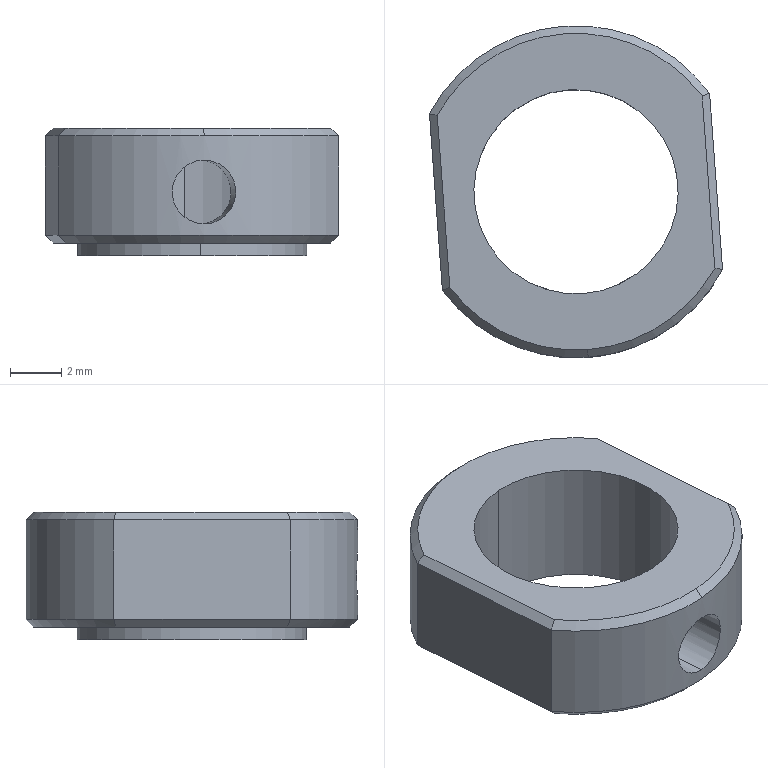Component | SolidWorks | MotorAssemblyWhen2-1_M8Nut2-1 | 1 solid | 24 faces | box 11.48 x 13 x 5 mm | volume 320 mm3 | cylinder 9 | plane 9 | cone 6 | commonest cylinder face diameters 13 x3 8 x2 2.5 x2 9 x2
STEP:
#1=COLOUR_RGB('',0.7922,0.8196,0.9333);
#2=FILL_AREA_STYLE_COLOUR('',#1);
#3=FILL_AREA_STYLE('',(#2));
#4=SURFACE_STYLE_FILL_AREA(#3);
#5=SURFACE_SIDE_STYLE('',(#4));
#6=SURFACE_STYLE_USAGE(.BOTH.,#5);
#7=PRESENTATION_STYLE_ASSIGNMENT((#6));
#8=CARTESIAN_POINT('',(-1.98,5.492,-5.202));
#9=VERTEX_POINT('',#8);
#10=CARTESIAN_POINT('',(-1.957,5.178,-5.202));
#11=VERTEX_POINT('',#10);
#12=CARTESIAN_POINT('',(-1.969,5.335,-5.202));
#13=DIRECTION('',(-0.,0.,-1.));
#14=DIRECTION('',(0.07337,-0.9973,0.));
#15=AXIS2_PLACEMENT_3D('',#12,#13,#14);
#16=CIRCLE('',#15,0.1575);
#17=EDGE_CURVE('',#9,#11,#16,.T.);
#18=ORIENTED_EDGE('',*,*,#17,.F.);
#19=CARTESIAN_POINT('',(-1.98,5.492,-5.398));
#20=VERTEX_POINT('',#19);
#21=CARTESIAN_POINT('',(-1.98,5.492,-5.202));
#22=DIRECTION('',(-0.,0.,-1.));
#23=VECTOR('',#22,39.37);
#24=LINE('',#21,#23);
#25=EDGE_CURVE('',#9,#20,#24,.T.);
#26=ORIENTED_EDGE('',*,*,#25,.T.);
#27=CARTESIAN_POINT('',(-1.957,5.178,-5.398));
#28=VERTEX_POINT('',#27);
#29=CARTESIAN_POINT('',(-1.969,5.335,-5.398));
#30=DIRECTION('',(-0.,0.,-1.));
#31=DIRECTION('',(0.07337,-0.9973,0.));
#32=AXIS2_PLACEMENT_3D('',#29,#30,#31);
#33=CIRCLE('',#32,0.1575);
#34=EDGE_CURVE('',#20,#28,#33,.T.);
#35=ORIENTED_EDGE('',*,*,#34,.T.);
#36=CARTESIAN_POINT('',(-1.957,5.178,-5.349));
#37=VERTEX_POINT('',#36);
#38=CARTESIAN_POINT('',(-1.957,5.178,-5.202));
#39=DIRECTION('',(-0.,0.,-1.));
#40=VECTOR('',#39,39.37);
#41=LINE('',#38,#40);
#42=EDGE_CURVE('',#37,#28,#41,.T.);
#43=ORIENTED_EDGE('',*,*,#42,.F.);
#44=CARTESIAN_POINT('',(-1.957,5.178,-5.251));
#45=VERTEX_POINT('',#44);
#46=CARTESIAN_POINT('',(-1.957,5.178,-5.251));
#47=CARTESIAN_POINT('',(-1.95,5.178,-5.251));
#48=CARTESIAN_POINT('',(-1.944,5.179,-5.252));
#49=CARTESIAN_POINT('',(-1.932,5.181,-5.257));
#50=CARTESIAN_POINT('',(-1.927,5.183,-5.261));
#51=CARTESIAN_POINT('',(-1.918,5.185,-5.27));
#52=CARTESIAN_POINT('',(-1.915,5.187,-5.275));
#53=CARTESIAN_POINT('',(-1.91,5.189,-5.287));
#54=CARTESIAN_POINT('',(-1.908,5.189,-5.294));
#55=CARTESIAN_POINT('',(-1.908,5.189,-5.303));
#56=CARTESIAN_POINT('',(-1.909,5.189,-5.307));
#57=CARTESIAN_POINT('',(-1.91,5.188,-5.313));
#58=CARTESIAN_POINT('',(-1.911,5.188,-5.316));
#59=CARTESIAN_POINT('',(-1.915,5.187,-5.325));
#60=CARTESIAN_POINT('',(-1.918,5.185,-5.33));
#61=CARTESIAN_POINT('',(-1.925,5.183,-5.337));
#62=CARTESIAN_POINT('',(-1.927,5.183,-5.339));
#63=CARTESIAN_POINT('',(-1.932,5.181,-5.343));
#64=CARTESIAN_POINT('',(-1.935,5.181,-5.344));
#65=CARTESIAN_POINT('',(-1.944,5.179,-5.348));
#66=CARTESIAN_POINT('',(-1.951,5.178,-5.349));
#67=CARTESIAN_POINT('',(-1.957,5.178,-5.349));
#68=B_SPLINE_CURVE_WITH_KNOTS('',3,(#46,#47,#48,#49,#50,#51,#52,#53,#54,#55,#56,#57,#58,#59,#60,#61,#62,#63,#64,#65,#66,#67),.UNSPECIFIED.,.F.,.F.,(4,2,2,2,2,2,2,2,2,2,4),(0.,0.0004916,0.0009832,0.001475,0.001966,0.002212,0.002458,0.00295,0.003195,0.003441,0.003933),.UNSPECIFIED.);
#69=EDGE_CURVE('',#45,#37,#68,.T.);
#70=ORIENTED_EDGE('',*,*,#69,.F.);
#71=CARTESIAN_POINT('',(-1.957,5.178,-5.202));
#72=DIRECTION('',(-0.,0.,-1.));
#73=VECTOR('',#72,39.37);
#74=LINE('',#71,#73);
#75=EDGE_CURVE('',#11,#45,#74,.T.);
#76=ORIENTED_EDGE('',*,*,#75,.F.);
#77=EDGE_LOOP('',(#18,#26,#35,#43,#70,#76));
#78=FACE_OUTER_BOUND('',#77,.T.);
#79=CARTESIAN_POINT('',(-1.969,5.335,-5.202));
#80=DIRECTION('',(-0.,0.,-1.));
#81=DIRECTION('',(0.07337,-0.9973,0.));
#82=AXIS2_PLACEMENT_3D('',#79,#80,#81);
#83=CYLINDRICAL_SURFACE('',#82,0.1575);
#84=ADVANCED_FACE('',(#78),#83,.F.);
#85=CARTESIAN_POINT('',(-1.986,5.578,-5.379));
#86=VERTEX_POINT('',#85);
#87=CARTESIAN_POINT('',(-1.774,5.482,-5.379));
#88=VERTEX_POINT('',#87);
#89=CARTESIAN_POINT('',(-1.969,5.335,-5.379));
#90=DIRECTION('',(-0.,0.,-1.));
#91=DIRECTION('',(0.07337,-0.9973,0.));
#92=AXIS2_PLACEMENT_3D('',#89,#90,#91);
#93=CIRCLE('',#92,0.2441);
#94=EDGE_CURVE('',#86,#88,#93,.T.);
#95=ORIENTED_EDGE('',*,*,#94,.F.);
#96=CARTESIAN_POINT('',(-1.987,5.59,-5.367));
#97=VERTEX_POINT('',#96);
#98=CARTESIAN_POINT('',(-1.987,5.59,-5.367));
#99=DIRECTION('',(-0.05188,0.7052,0.7071));
#100=VECTOR('',#99,39.37);
#101=LINE('',#98,#100);
#102=EDGE_CURVE('',#86,#97,#101,.T.);
#103=ORIENTED_EDGE('',*,*,#102,.T.);
#104=CARTESIAN_POINT('',(-1.763,5.487,-5.367));
#105=VERTEX_POINT('',#104);
#106=CARTESIAN_POINT('',(-1.969,5.335,-5.367));
#107=DIRECTION('',(0.,-0.,1.));
#108=DIRECTION('',(0.07337,-0.9973,0.));
#109=AXIS2_PLACEMENT_3D('',#106,#107,#108);
#110=CIRCLE('',#109,0.2559);
#111=EDGE_CURVE('',#105,#97,#110,.T.);
#112=ORIENTED_EDGE('',*,*,#111,.F.);
#113=CARTESIAN_POINT('',(-1.774,5.482,-5.379));
#114=CARTESIAN_POINT('',(-1.77,5.484,-5.375));
#115=CARTESIAN_POINT('',(-1.766,5.485,-5.371));
#116=CARTESIAN_POINT('',(-1.763,5.487,-5.367));
#117=B_SPLINE_CURVE_WITH_KNOTS('',3,(#113,#114,#115,#116),.UNSPECIFIED.,.F.,.F.,(4,4),(0.,0.0004332),.UNSPECIFIED.);
#118=EDGE_CURVE('',#88,#105,#117,.T.);
#119=ORIENTED_EDGE('',*,*,#118,.F.);
#120=EDGE_LOOP('',(#95,#103,#112,#119));
#121=FACE_OUTER_BOUND('',#120,.T.);
#122=CARTESIAN_POINT('',(-1.969,5.335,-5.367));
#123=DIRECTION('',(0.,-0.,1.));
#124=DIRECTION('',(-0.07337,0.9973,0.));
#125=AXIS2_PLACEMENT_3D('',#122,#123,#124);
#126=CONICAL_SURFACE('',#125,0.2559,0.7854);
#127=ADVANCED_FACE('',(#121),#126,.T.);
#128=CARTESIAN_POINT('',(-1.951,5.091,-5.202));
#129=VERTEX_POINT('',#128);
#130=CARTESIAN_POINT('',(-1.755,5.217,-5.202));
#131=VERTEX_POINT('',#130);
#132=CARTESIAN_POINT('',(-1.969,5.335,-5.202));
#133=DIRECTION('',(0.,-0.,1.));
#134=DIRECTION('',(0.07337,-0.9973,0.));
#135=AXIS2_PLACEMENT_3D('',#132,#133,#134);
#136=CIRCLE('',#135,0.2441);
#137=EDGE_CURVE('',#129,#131,#136,.T.);
#138=ORIENTED_EDGE('',*,*,#137,.F.);
#139=CARTESIAN_POINT('',(-1.95,5.079,-5.213));
#140=VERTEX_POINT('',#139);
#141=CARTESIAN_POINT('',(-1.95,5.079,-5.213));
#142=DIRECTION('',(0.05188,-0.7052,-0.7071));
#143=VECTOR('',#142,39.37);
#144=LINE('',#141,#143);
#145=EDGE_CURVE('',#129,#140,#144,.T.);
#146=ORIENTED_EDGE('',*,*,#145,.T.);
#147=CARTESIAN_POINT('',(-1.743,5.215,-5.213));
#148=VERTEX_POINT('',#147);
#149=CARTESIAN_POINT('',(-1.969,5.335,-5.213));
#150=DIRECTION('',(-0.,0.,-1.));
#151=DIRECTION('',(0.07337,-0.9973,0.));
#152=AXIS2_PLACEMENT_3D('',#149,#150,#151);
#153=CIRCLE('',#152,0.2559);
#154=EDGE_CURVE('',#148,#140,#153,.T.);
#155=ORIENTED_EDGE('',*,*,#154,.F.);
#156=CARTESIAN_POINT('',(-1.743,5.215,-5.213));
#157=CARTESIAN_POINT('',(-1.747,5.215,-5.209));
#158=CARTESIAN_POINT('',(-1.751,5.216,-5.206));
#159=CARTESIAN_POINT('',(-1.755,5.217,-5.202));
#160=B_SPLINE_CURVE_WITH_KNOTS('',3,(#156,#157,#158,#159),.UNSPECIFIED.,.F.,.F.,(4,4),(0.,0.0004332),.UNSPECIFIED.);
#161=EDGE_CURVE('',#148,#131,#160,.T.);
#162=ORIENTED_EDGE('',*,*,#161,.T.);
#163=EDGE_LOOP('',(#138,#146,#155,#162));
#164=FACE_OUTER_BOUND('',#163,.T.);
#165=CARTESIAN_POINT('',(-1.969,5.335,-5.213));
#166=DIRECTION('',(-0.,0.,-1.));
#167=DIRECTION('',(0.07337,-0.9973,0.));
#168=AXIS2_PLACEMENT_3D('',#165,#166,#167);
#169=CONICAL_SURFACE('',#168,0.2559,0.7854);
#170=ADVANCED_FACE('',(#164),#169,.T.);
#171=ORIENTED_EDGE('',*,*,#111,.T.);
#172=CARTESIAN_POINT('',(-1.987,5.59,-5.213));
#173=VERTEX_POINT('',#172);
#174=CARTESIAN_POINT('',(-1.987,5.59,-5.398));
#175=DIRECTION('',(0.,-0.,1.));
#176=VECTOR('',#175,39.37);
#177=LINE('',#174,#176);
#178=EDGE_CURVE('',#97,#173,#177,.T.);
#179=ORIENTED_EDGE('',*,*,#178,.T.);
#180=CARTESIAN_POINT('',(-1.763,5.487,-5.213));
#181=VERTEX_POINT('',#180);
#182=CARTESIAN_POINT('',(-1.969,5.335,-5.213));
#183=DIRECTION('',(-0.,0.,-1.));
#184=DIRECTION('',(0.07337,-0.9973,0.));
#185=AXIS2_PLACEMENT_3D('',#182,#183,#184);
#186=CIRCLE('',#185,0.2559);
#187=EDGE_CURVE('',#173,#181,#186,.T.);
#188=ORIENTED_EDGE('',*,*,#187,.T.);
#189=CARTESIAN_POINT('',(-1.763,5.487,-5.202));
#190=DIRECTION('',(0.,-0.,1.));
#191=VECTOR('',#190,39.37);
#192=LINE('',#189,#191);
#193=EDGE_CURVE('',#105,#181,#192,.T.);
#194=ORIENTED_EDGE('',*,*,#193,.F.);
#195=EDGE_LOOP('',(#171,#179,#188,#194));
#196=FACE_OUTER_BOUND('',#195,.T.);
#197=CARTESIAN_POINT('',(-1.969,5.335,-5.398));
#198=DIRECTION('',(0.,-0.,1.));
#199=DIRECTION('',(-0.07337,0.9973,0.));
#200=AXIS2_PLACEMENT_3D('',#197,#198,#199);
#201=CYLINDRICAL_SURFACE('',#200,0.2559);
#202=ADVANCED_FACE('',(#196),#201,.T.);
#203=ORIENTED_EDGE('',*,*,#69,.T.);
#204=CARTESIAN_POINT('',(-1.95,5.079,-5.349));
#205=VERTEX_POINT('',#204);
#206=CARTESIAN_POINT('',(-1.945,5.021,-5.349));
#207=DIRECTION('',(0.07337,-0.9973,-0.));
#208=VECTOR('',#207,39.37);
#209=LINE('',#206,#208);
#210=EDGE_CURVE('',#37,#205,#209,.T.);
#211=ORIENTED_EDGE('',*,*,#210,.T.);
#212=CARTESIAN_POINT('',(-1.95,5.079,-5.251));
#213=VERTEX_POINT('',#212);
#214=CARTESIAN_POINT('',(-1.95,5.079,-5.251));
#215=CARTESIAN_POINT('',(-1.943,5.08,-5.251));
#216=CARTESIAN_POINT('',(-1.937,5.081,-5.252));
#217=CARTESIAN_POINT('',(-1.925,5.082,-5.257));
#218=CARTESIAN_POINT('',(-1.92,5.083,-5.261));
#219=CARTESIAN_POINT('',(-1.911,5.085,-5.27));
#220=CARTESIAN_POINT('',(-1.907,5.086,-5.275));
#221=CARTESIAN_POINT('',(-1.902,5.087,-5.287));
#222=CARTESIAN_POINT('',(-1.901,5.088,-5.294));
#223=CARTESIAN_POINT('',(-1.901,5.088,-5.303));
#224=CARTESIAN_POINT('',(-1.901,5.088,-5.306));
#225=CARTESIAN_POINT('',(-1.903,5.087,-5.313));
#226=CARTESIAN_POINT('',(-1.903,5.087,-5.316));
#227=CARTESIAN_POINT('',(-1.907,5.086,-5.325));
#228=CARTESIAN_POINT('',(-1.911,5.085,-5.33));
#229=CARTESIAN_POINT('',(-1.92,5.083,-5.339));
#230=CARTESIAN_POINT('',(-1.925,5.082,-5.343));
#231=CARTESIAN_POINT('',(-1.937,5.081,-5.348));
#232=CARTESIAN_POINT('',(-1.943,5.08,-5.349));
#233=CARTESIAN_POINT('',(-1.95,5.079,-5.349));
#234=B_SPLINE_CURVE_WITH_KNOTS('',3,(#214,#215,#216,#217,#218,#219,#220,#221,#222,#223,#224,#225,#226,#227,#228,#229,#230,#231,#232,#233),.UNSPECIFIED.,.F.,.F.,(4,2,2,2,2,2,2,2,2,4),(0.003916,0.004406,0.004895,0.005385,0.005874,0.006119,0.006364,0.006853,0.007343,0.007832),.UNSPECIFIED.);
#235=EDGE_CURVE('',#213,#205,#234,.T.);
#236=ORIENTED_EDGE('',*,*,#235,.F.);
#237=CARTESIAN_POINT('',(-1.945,5.021,-5.251));
#238=DIRECTION('',(0.07337,-0.9973,-0.));
#239=VECTOR('',#238,39.37);
#240=LINE('',#237,#239);
#241=EDGE_CURVE('',#45,#213,#240,.T.);
#242=ORIENTED_EDGE('',*,*,#241,.F.);
#243=EDGE_LOOP('',(#203,#211,#236,#242));
#244=FACE_OUTER_BOUND('',#243,.T.);
#245=CARTESIAN_POINT('',(-1.945,5.021,-5.3));
#246=DIRECTION('',(0.07337,-0.9973,-0.));
#247=DIRECTION('',(0.,0.,1.));
#248=AXIS2_PLACEMENT_3D('',#245,#246,#247);
#249=CYLINDRICAL_SURFACE('',#248,0.04921);
#250=ADVANCED_FACE('',(#244),#249,.F.);
#251=CARTESIAN_POINT('',(-1.982,5.511,-5.379));
#252=VERTEX_POINT('',#251);
#253=CARTESIAN_POINT('',(-1.956,5.158,-5.379));
#254=VERTEX_POINT('',#253);
#255=CARTESIAN_POINT('',(-1.969,5.335,-5.379));
#256=DIRECTION('',(0.,-0.,1.));
#257=DIRECTION('',(0.07337,-0.9973,0.));
#258=AXIS2_PLACEMENT_3D('',#255,#256,#257);
#259=CIRCLE('',#258,0.1772);
#260=EDGE_CURVE('',#252,#254,#259,.T.);
#261=ORIENTED_EDGE('',*,*,#260,.F.);
#262=CARTESIAN_POINT('',(-1.982,5.511,-5.398));
#263=VERTEX_POINT('',#262);
#264=CARTESIAN_POINT('',(-1.982,5.511,-5.379));
#265=DIRECTION('',(-0.,0.,-1.));
#266=VECTOR('',#265,39.37);
#267=LINE('',#264,#266);
#268=EDGE_CURVE('',#252,#263,#267,.T.);
#269=ORIENTED_EDGE('',*,*,#268,.T.);
#270=CARTESIAN_POINT('',(-1.956,5.158,-5.398));
#271=VERTEX_POINT('',#270);
#272=CARTESIAN_POINT('',(-1.969,5.335,-5.398));
#273=DIRECTION('',(-0.,0.,-1.));
#274=DIRECTION('',(0.07337,-0.9973,0.));
#275=AXIS2_PLACEMENT_3D('',#272,#273,#274);
#276=CIRCLE('',#275,0.1772);
#277=EDGE_CURVE('',#271,#263,#276,.T.);
#278=ORIENTED_EDGE('',*,*,#277,.F.);
#279=CARTESIAN_POINT('',(-1.956,5.158,-5.379));
#280=DIRECTION('',(-0.,0.,-1.));
#281=VECTOR('',#280,39.37);
#282=LINE('',#279,#281);
#283=EDGE_CURVE('',#254,#271,#282,.T.);
#284=ORIENTED_EDGE('',*,*,#283,.F.);
#285=EDGE_LOOP('',(#261,#269,#278,#284));
#286=FACE_OUTER_BOUND('',#285,.T.);
#287=CARTESIAN_POINT('',(-1.969,5.335,-5.379));
#288=DIRECTION('',(-0.,0.,-1.));
#289=DIRECTION('',(0.07337,-0.9973,0.));
#290=AXIS2_PLACEMENT_3D('',#287,#288,#289);
#291=CYLINDRICAL_SURFACE('',#290,0.1772);
#292=ADVANCED_FACE('',(#286),#291,.T.);
#293=CARTESIAN_POINT('',(-1.969,5.335,-5.202));
#294=DIRECTION('',(-0.,0.,-1.));
#295=DIRECTION('',(0.07337,-0.9973,0.));
#296=AXIS2_PLACEMENT_3D('',#293,#294,#295);
#297=CIRCLE('',#296,0.1575);
#298=EDGE_CURVE('',#11,#9,#297,.T.);
#299=ORIENTED_EDGE('',*,*,#298,.T.);
#300=ORIENTED_EDGE('',*,*,#17,.T.);
#301=EDGE_LOOP('',(#299,#300));
#302=FACE_BOUND('',#301,.T.);
#303=CARTESIAN_POINT('',(-1.774,5.482,-5.202));
#304=VERTEX_POINT('',#303);
#305=CARTESIAN_POINT('',(-2.182,5.452,-5.202));
#306=VERTEX_POINT('',#305);
#307=CARTESIAN_POINT('',(-1.969,5.335,-5.202));
#308=DIRECTION('',(0.,-0.,1.));
#309=DIRECTION('',(0.07337,-0.9973,0.));
#310=AXIS2_PLACEMENT_3D('',#307,#308,#309);
#311=CIRCLE('',#310,0.2441);
#312=EDGE_CURVE('',#304,#306,#311,.T.);
#313=ORIENTED_EDGE('',*,*,#312,.T.);
#314=CARTESIAN_POINT('',(-2.163,5.187,-5.202));
#315=VERTEX_POINT('',#314);
#316=CARTESIAN_POINT('',(-2.163,5.184,-5.202));
#317=DIRECTION('',(0.07337,-0.9973,-0.));
#318=VECTOR('',#317,39.37);
#319=LINE('',#316,#318);
#320=EDGE_CURVE('',#306,#315,#319,.T.);
#321=ORIENTED_EDGE('',*,*,#320,.T.);
#322=CARTESIAN_POINT('',(-1.969,5.335,-5.202));
#323=DIRECTION('',(0.,-0.,1.));
#324=DIRECTION('',(0.07337,-0.9973,0.));
#325=AXIS2_PLACEMENT_3D('',#322,#323,#324);
#326=CIRCLE('',#325,0.2441);
#327=EDGE_CURVE('',#315,#129,#326,.T.);
#328=ORIENTED_EDGE('',*,*,#327,.T.);
#329=ORIENTED_EDGE('',*,*,#137,.T.);
#330=CARTESIAN_POINT('',(-1.774,5.486,-5.202));
#331=DIRECTION('',(-0.07337,0.9973,0.));
#332=VECTOR('',#331,39.37);
#333=LINE('',#330,#332);
#334=EDGE_CURVE('',#131,#304,#333,.T.);
#335=ORIENTED_EDGE('',*,*,#334,.T.);
#336=EDGE_LOOP('',(#313,#321,#328,#329,#335));
#337=FACE_OUTER_BOUND('',#336,.T.);
#338=CARTESIAN_POINT('',(-1.969,5.335,-5.202));
#339=DIRECTION('',(-0.,0.,-1.));
#340=DIRECTION('',(0.07337,-0.9973,-0.));
#341=AXIS2_PLACEMENT_3D('',#338,#339,#340);
#342=PLANE('',#341);
#343=ADVANCED_FACE('',(#302,#337),#342,.F.);
#344=ORIENTED_EDGE('',*,*,#193,.T.);
#345=CARTESIAN_POINT('',(-1.743,5.215,-5.213));
#346=DIRECTION('',(0.07337,-0.9973,-0.));
#347=VECTOR('',#346,39.37);
#348=LINE('',#345,#347);
#349=EDGE_CURVE('',#181,#148,#348,.T.);
#350=ORIENTED_EDGE('',*,*,#349,.T.);
#351=CARTESIAN_POINT('',(-1.743,5.215,-5.367));
#352=VERTEX_POINT('',#351);
#353=CARTESIAN_POINT('',(-1.743,5.215,-5.202));
#354=DIRECTION('',(-0.,0.,-1.));
#355=VECTOR('',#354,39.37);
#356=LINE('',#353,#355);
#357=EDGE_CURVE('',#148,#352,#356,.T.);
#358=ORIENTED_EDGE('',*,*,#357,.T.);
#359=CARTESIAN_POINT('',(-1.781,5.743,-5.367));
#360=DIRECTION('',(-0.07337,0.9973,0.));
#361=VECTOR('',#360,39.37);
#362=LINE('',#359,#361);
#363=EDGE_CURVE('',#352,#105,#362,.T.);
#364=ORIENTED_EDGE('',*,*,#363,.T.);
#365=EDGE_LOOP('',(#344,#350,#358,#364));
#366=FACE_OUTER_BOUND('',#365,.T.);
#367=CARTESIAN_POINT('',(-1.781,5.743,-5.202));
#368=DIRECTION('',(0.9973,0.07337,0.));
#369=DIRECTION('',(0.,-0.,1.));
#370=AXIS2_PLACEMENT_3D('',#367,#368,#369);
#371=PLANE('',#370);
#372=ADVANCED_FACE('',(#366),#371,.T.);
#373=ORIENTED_EDGE('',*,*,#178,.F.);
#374=CARTESIAN_POINT('',(-2.194,5.455,-5.367));
#375=VERTEX_POINT('',#374);
#376=CARTESIAN_POINT('',(-1.969,5.335,-5.367));
#377=DIRECTION('',(0.,-0.,1.));
#378=DIRECTION('',(0.07337,-0.9973,0.));
#379=AXIS2_PLACEMENT_3D('',#376,#377,#378);
#380=CIRCLE('',#379,0.2559);
#381=EDGE_CURVE('',#97,#375,#380,.T.);
#382=ORIENTED_EDGE('',*,*,#381,.T.);
#383=CARTESIAN_POINT('',(-2.194,5.455,-5.213));
#384=VERTEX_POINT('',#383);
#385=CARTESIAN_POINT('',(-2.194,5.455,-5.398));
#386=DIRECTION('',(0.,-0.,1.));
#387=VECTOR('',#386,39.37);
#388=LINE('',#385,#387);
#389=EDGE_CURVE('',#375,#384,#388,.T.);
#390=ORIENTED_EDGE('',*,*,#389,.T.);
#391=CARTESIAN_POINT('',(-1.969,5.335,-5.213));
#392=DIRECTION('',(-0.,0.,-1.));
#393=DIRECTION('',(0.07337,-0.9973,0.));
#394=AXIS2_PLACEMENT_3D('',#391,#392,#393);
#395=CIRCLE('',#394,0.2559);
#396=EDGE_CURVE('',#384,#173,#395,.T.);
#397=ORIENTED_EDGE('',*,*,#396,.T.);
#398=EDGE_LOOP('',(#373,#382,#390,#397));
#399=FACE_OUTER_BOUND('',#398,.T.);
#400=CARTESIAN_POINT('',(-1.969,5.335,-5.398));
#401=DIRECTION('',(0.,-0.,1.));
#402=DIRECTION('',(-0.07337,0.9973,0.));
#403=AXIS2_PLACEMENT_3D('',#400,#401,#402);
#404=CYLINDRICAL_SURFACE('',#403,0.2559);
#405=ADVANCED_FACE('',(#399),#404,.T.);
#406=CARTESIAN_POINT('',(-2.174,5.183,-5.367));
#407=VERTEX_POINT('',#406);
#408=CARTESIAN_POINT('',(-2.174,5.183,-5.213));
#409=VERTEX_POINT('',#408);
#410=CARTESIAN_POINT('',(-2.174,5.183,-5.202));
#411=DIRECTION('',(0.,-0.,1.));
#412=VECTOR('',#411,39.37);
#413=LINE('',#410,#412);
#414=EDGE_CURVE('',#407,#409,#413,.T.);
#415=ORIENTED_EDGE('',*,*,#414,.T.);
#416=CARTESIAN_POINT('',(-2.194,5.455,-5.213));
#417=DIRECTION('',(-0.07337,0.9973,0.));
#418=VECTOR('',#417,39.37);
#419=LINE('',#416,#418);
#420=EDGE_CURVE('',#409,#384,#419,.T.);
#421=ORIENTED_EDGE('',*,*,#420,.T.);
#422=ORIENTED_EDGE('',*,*,#389,.F.);
#423=CARTESIAN_POINT('',(-2.213,5.711,-5.367));
#424=DIRECTION('',(0.07337,-0.9973,-0.));
#425=VECTOR('',#424,39.37);
#426=LINE('',#423,#425);
#427=EDGE_CURVE('',#375,#407,#426,.T.);
#428=ORIENTED_EDGE('',*,*,#427,.T.);
#429=EDGE_LOOP('',(#415,#421,#422,#428));
#430=FACE_OUTER_BOUND('',#429,.T.);
#431=CARTESIAN_POINT('',(-2.213,5.711,-5.202));
#432=DIRECTION('',(-0.9973,-0.07337,-0.));
#433=DIRECTION('',(-0.,0.,-1.));
#434=AXIS2_PLACEMENT_3D('',#431,#432,#433);
#435=PLANE('',#434);
#436=ADVANCED_FACE('',(#430),#435,.T.);
#437=ORIENTED_EDGE('',*,*,#357,.F.);
#438=ORIENTED_EDGE('',*,*,#154,.T.);
#439=CARTESIAN_POINT('',(-1.969,5.335,-5.213));
#440=DIRECTION('',(-0.,0.,-1.));
#441=DIRECTION('',(0.07337,-0.9973,0.));
#442=AXIS2_PLACEMENT_3D('',#439,#440,#441);
#443=CIRCLE('',#442,0.2559);
#444=EDGE_CURVE('',#140,#409,#443,.T.);
#445=ORIENTED_EDGE('',*,*,#444,.T.);
#446=ORIENTED_EDGE('',*,*,#414,.F.);
#447=CARTESIAN_POINT('',(-1.969,5.335,-5.367));
#448=DIRECTION('',(0.,-0.,1.));
#449=DIRECTION('',(0.07337,-0.9973,0.));
#450=AXIS2_PLACEMENT_3D('',#447,#448,#449);
#451=CIRCLE('',#450,0.2559);
#452=EDGE_CURVE('',#407,#352,#451,.T.);
#453=ORIENTED_EDGE('',*,*,#452,.T.);
#454=EDGE_LOOP('',(#437,#438,#445,#446,#453));
#455=FACE_OUTER_BOUND('',#454,.T.);
#456=ORIENTED_EDGE('',*,*,#235,.T.);
#457=CARTESIAN_POINT('',(-1.95,5.079,-5.349));
#458=CARTESIAN_POINT('',(-1.956,5.079,-5.349));
#459=CARTESIAN_POINT('',(-1.963,5.079,-5.348));
#460=CARTESIAN_POINT('',(-1.975,5.079,-5.343));
#461=CARTESIAN_POINT('',(-1.98,5.079,-5.339));
#462=CARTESIAN_POINT('',(-1.989,5.08,-5.33));
#463=CARTESIAN_POINT('',(-1.993,5.08,-5.325));
#464=CARTESIAN_POINT('',(-1.998,5.08,-5.313));
#465=CARTESIAN_POINT('',(-1.999,5.081,-5.307));
#466=CARTESIAN_POINT('',(-1.999,5.081,-5.297));
#467=CARTESIAN_POINT('',(-1.999,5.081,-5.294));
#468=CARTESIAN_POINT('',(-1.998,5.08,-5.287));
#469=CARTESIAN_POINT('',(-1.997,5.08,-5.284));
#470=CARTESIAN_POINT('',(-1.993,5.08,-5.275));
#471=CARTESIAN_POINT('',(-1.989,5.08,-5.27));
#472=CARTESIAN_POINT('',(-1.98,5.079,-5.261));
#473=CARTESIAN_POINT('',(-1.975,5.079,-5.257));
#474=CARTESIAN_POINT('',(-1.963,5.079,-5.252));
#475=CARTESIAN_POINT('',(-1.956,5.079,-5.251));
#476=CARTESIAN_POINT('',(-1.95,5.079,-5.251));
#477=B_SPLINE_CURVE_WITH_KNOTS('',3,(#457,#458,#459,#460,#461,#462,#463,#464,#465,#466,#467,#468,#469,#470,#471,#472,#473,#474,#475,#476),.UNSPECIFIED.,.F.,.F.,(4,2,2,2,2,2,2,2,2,4),(0.,0.0004895,0.000979,0.001469,0.001958,0.002203,0.002448,0.002937,0.003427,0.003916),.UNSPECIFIED.);
#478=EDGE_CURVE('',#205,#213,#477,.T.);
#479=ORIENTED_EDGE('',*,*,#478,.T.);
#480=EDGE_LOOP('',(#456,#479));
#481=FACE_BOUND('',#480,.T.);
#482=CARTESIAN_POINT('',(-1.969,5.335,-5.398));
#483=DIRECTION('',(0.,-0.,1.));
#484=DIRECTION('',(-0.07337,0.9973,0.));
#485=AXIS2_PLACEMENT_3D('',#482,#483,#484);
#486=CYLINDRICAL_SURFACE('',#485,0.2559);
#487=ADVANCED_FACE('',(#455,#481),#486,.T.);
#488=CARTESIAN_POINT('',(-2.182,5.452,-5.379));
#489=VERTEX_POINT('',#488);
#490=CARTESIAN_POINT('',(-1.969,5.335,-5.379));
#491=DIRECTION('',(-0.,0.,-1.));
#492=DIRECTION('',(0.07337,-0.9973,0.));
#493=AXIS2_PLACEMENT_3D('',#490,#491,#492);
#494=CIRCLE('',#493,0.2441);
#495=EDGE_CURVE('',#489,#86,#494,.T.);
#496=ORIENTED_EDGE('',*,*,#495,.T.);
#497=ORIENTED_EDGE('',*,*,#94,.T.);
#498=CARTESIAN_POINT('',(-1.755,5.217,-5.379));
#499=VERTEX_POINT('',#498);
#500=CARTESIAN_POINT('',(-1.764,5.35,-5.379));
#501=DIRECTION('',(0.07337,-0.9973,-0.));
#502=VECTOR('',#501,39.37);
#503=LINE('',#500,#502);
#504=EDGE_CURVE('',#88,#499,#503,.T.);
#505=ORIENTED_EDGE('',*,*,#504,.T.);
#506=CARTESIAN_POINT('',(-2.163,5.187,-5.379));
#507=VERTEX_POINT('',#506);
#508=CARTESIAN_POINT('',(-1.969,5.335,-5.379));
#509=DIRECTION('',(-0.,0.,-1.));
#510=DIRECTION('',(0.07337,-0.9973,0.));
#511=AXIS2_PLACEMENT_3D('',#508,#509,#510);
#512=CIRCLE('',#511,0.2441);
#513=EDGE_CURVE('',#499,#507,#512,.T.);
#514=ORIENTED_EDGE('',*,*,#513,.T.);
#515=CARTESIAN_POINT('',(-2.173,5.32,-5.379));
#516=DIRECTION('',(-0.07337,0.9973,0.));
#517=VECTOR('',#516,39.37);
#518=LINE('',#515,#517);
#519=EDGE_CURVE('',#507,#489,#518,.T.);
#520=ORIENTED_EDGE('',*,*,#519,.T.);
#521=EDGE_LOOP('',(#496,#497,#505,#514,#520));
#522=FACE_OUTER_BOUND('',#521,.T.);
#523=CARTESIAN_POINT('',(-1.969,5.335,-5.379));
#524=DIRECTION('',(0.,-0.,1.));
#525=DIRECTION('',(0.07337,-0.9973,0.));
#526=AXIS2_PLACEMENT_3D('',#523,#524,#525);
#527=CIRCLE('',#526,0.1772);
#528=EDGE_CURVE('',#254,#252,#527,.T.);
#529=ORIENTED_EDGE('',*,*,#528,.T.);
#530=ORIENTED_EDGE('',*,*,#260,.T.);
#531=EDGE_LOOP('',(#529,#530));
#532=FACE_BOUND('',#531,.T.);
#533=CARTESIAN_POINT('',(-1.969,5.335,-5.379));
#534=DIRECTION('',(-0.,0.,-1.));
#535=DIRECTION('',(0.07337,-0.9973,-0.));
#536=AXIS2_PLACEMENT_3D('',#533,#534,#535);
#537=PLANE('',#536);
#538=ADVANCED_FACE('',(#522,#532),#537,.T.);
#539=ORIENTED_EDGE('',*,*,#210,.F.);
#540=CARTESIAN_POINT('',(-1.957,5.178,-5.349));
#541=CARTESIAN_POINT('',(-1.963,5.177,-5.349));
#542=CARTESIAN_POINT('',(-1.97,5.177,-5.348));
#543=CARTESIAN_POINT('',(-1.982,5.178,-5.343));
#544=CARTESIAN_POINT('',(-1.987,5.178,-5.339));
#545=CARTESIAN_POINT('',(-1.997,5.18,-5.33));
#546=CARTESIAN_POINT('',(-2.,5.18,-5.325));
#547=CARTESIAN_POINT('',(-2.004,5.181,-5.316));
#548=CARTESIAN_POINT('',(-2.005,5.181,-5.313));
#549=CARTESIAN_POINT('',(-2.006,5.182,-5.307));
#550=CARTESIAN_POINT('',(-2.007,5.182,-5.303));
#551=CARTESIAN_POINT('',(-2.007,5.182,-5.294));
#552=CARTESIAN_POINT('',(-2.005,5.181,-5.287));
#553=CARTESIAN_POINT('',(-2.,5.18,-5.275));
#554=CARTESIAN_POINT('',(-1.997,5.18,-5.27));
#555=CARTESIAN_POINT('',(-1.987,5.178,-5.261));
#556=CARTESIAN_POINT('',(-1.982,5.178,-5.257));
#557=CARTESIAN_POINT('',(-1.97,5.177,-5.252));
#558=CARTESIAN_POINT('',(-1.963,5.177,-5.251));
#559=CARTESIAN_POINT('',(-1.957,5.178,-5.251));
#560=B_SPLINE_CURVE_WITH_KNOTS('',3,(#540,#541,#542,#543,#544,#545,#546,#547,#548,#549,#550,#551,#552,#553,#554,#555,#556,#557,#558,#559),.UNSPECIFIED.,.F.,.F.,(4,2,2,2,2,2,2,2,2,4),(0.003933,0.004424,0.004916,0.005407,0.005653,0.005899,0.00639,0.006882,0.007373,0.007865),.UNSPECIFIED.);
#561=EDGE_CURVE('',#37,#45,#560,.T.);
#562=ORIENTED_EDGE('',*,*,#561,.T.);
#563=ORIENTED_EDGE('',*,*,#241,.T.);
#564=ORIENTED_EDGE('',*,*,#478,.F.);
#565=EDGE_LOOP('',(#539,#562,#563,#564));
#566=FACE_OUTER_BOUND('',#565,.T.);
#567=CARTESIAN_POINT('',(-1.945,5.021,-5.3));
#568=DIRECTION('',(0.07337,-0.9973,-0.));
#569=DIRECTION('',(0.,0.,1.));
#570=AXIS2_PLACEMENT_3D('',#567,#568,#569);
#571=CYLINDRICAL_SURFACE('',#570,0.04921);
#572=ADVANCED_FACE('',(#566),#571,.F.);
#573=CARTESIAN_POINT('',(-1.969,5.335,-5.398));
#574=DIRECTION('',(-0.,0.,-1.));
#575=DIRECTION('',(0.07337,-0.9973,0.));
#576=AXIS2_PLACEMENT_3D('',#573,#574,#575);
#577=CIRCLE('',#576,0.1575);
#578=EDGE_CURVE('',#28,#20,#577,.T.);
#579=ORIENTED_EDGE('',*,*,#578,.F.);
#580=ORIENTED_EDGE('',*,*,#34,.F.);
#581=EDGE_LOOP('',(#579,#580));
#582=FACE_BOUND('',#581,.T.);
#583=ORIENTED_EDGE('',*,*,#277,.T.);
#584=CARTESIAN_POINT('',(-1.969,5.335,-5.398));
#585=DIRECTION('',(-0.,0.,-1.));
#586=DIRECTION('',(0.07337,-0.9973,0.));
#587=AXIS2_PLACEMENT_3D('',#584,#585,#586);
#588=CIRCLE('',#587,0.1772);
#589=EDGE_CURVE('',#263,#271,#588,.T.);
#590=ORIENTED_EDGE('',*,*,#589,.T.);
#591=EDGE_LOOP('',(#583,#590));
#592=FACE_OUTER_BOUND('',#591,.T.);
#593=CARTESIAN_POINT('',(-1.969,5.335,-5.398));
#594=DIRECTION('',(-0.,0.,-1.));
#595=DIRECTION('',(0.07337,-0.9973,-0.));
#596=AXIS2_PLACEMENT_3D('',#593,#594,#595);
#597=PLANE('',#596);
#598=ADVANCED_FACE('',(#582,#592),#597,.T.);
#599=ORIENTED_EDGE('',*,*,#268,.F.);
#600=ORIENTED_EDGE('',*,*,#528,.F.);
#601=ORIENTED_EDGE('',*,*,#283,.T.);
#602=ORIENTED_EDGE('',*,*,#589,.F.);
#603=EDGE_LOOP('',(#599,#600,#601,#602));
#604=FACE_OUTER_BOUND('',#603,.T.);
#605=CARTESIAN_POINT('',(-1.969,5.335,-5.379));
#606=DIRECTION('',(-0.,0.,-1.));
#607=DIRECTION('',(0.07337,-0.9973,0.));
#608=AXIS2_PLACEMENT_3D('',#605,#606,#607);
#609=CYLINDRICAL_SURFACE('',#608,0.1772);
#610=ADVANCED_FACE('',(#604),#609,.T.);
#611=CARTESIAN_POINT('',(-1.774,5.482,-5.202));
#612=CARTESIAN_POINT('',(-1.77,5.484,-5.206));
#613=CARTESIAN_POINT('',(-1.766,5.485,-5.209));
#614=CARTESIAN_POINT('',(-1.763,5.487,-5.213));
#615=B_SPLINE_CURVE_WITH_KNOTS('',3,(#611,#612,#613,#614),.UNSPECIFIED.,.F.,.F.,(4,4),(0.,0.0004332),.UNSPECIFIED.);
#616=EDGE_CURVE('',#304,#181,#615,.T.);
#617=ORIENTED_EDGE('',*,*,#616,.F.);
#618=ORIENTED_EDGE('',*,*,#334,.F.);
#619=ORIENTED_EDGE('',*,*,#161,.F.);
#620=ORIENTED_EDGE('',*,*,#349,.F.);
#621=EDGE_LOOP('',(#617,#618,#619,#620));
#622=FACE_OUTER_BOUND('',#621,.T.);
#623=CARTESIAN_POINT('',(-1.781,5.743,-5.213));
#624=DIRECTION('',(0.7052,0.05188,0.7071));
#625=DIRECTION('',(-0.7052,-0.05188,0.7071));
#626=AXIS2_PLACEMENT_3D('',#623,#624,#625);
#627=PLANE('',#626);
#628=ADVANCED_FACE('',(#622),#627,.T.);
#629=ORIENTED_EDGE('',*,*,#145,.F.);
#630=ORIENTED_EDGE('',*,*,#327,.F.);
#631=CARTESIAN_POINT('',(-2.174,5.183,-5.213));
#632=CARTESIAN_POINT('',(-2.171,5.184,-5.209));
#633=CARTESIAN_POINT('',(-2.167,5.186,-5.206));
#634=CARTESIAN_POINT('',(-2.163,5.187,-5.202));
#635=B_SPLINE_CURVE_WITH_KNOTS('',3,(#631,#632,#633,#634),.UNSPECIFIED.,.F.,.F.,(4,4),(0.,0.0004332),.UNSPECIFIED.);
#636=EDGE_CURVE('',#409,#315,#635,.T.);
#637=ORIENTED_EDGE('',*,*,#636,.F.);
#638=ORIENTED_EDGE('',*,*,#444,.F.);
#639=EDGE_LOOP('',(#629,#630,#637,#638));
#640=FACE_OUTER_BOUND('',#639,.T.);
#641=CARTESIAN_POINT('',(-1.969,5.335,-5.213));
#642=DIRECTION('',(-0.,0.,-1.));
#643=DIRECTION('',(0.07337,-0.9973,0.));
#644=AXIS2_PLACEMENT_3D('',#641,#642,#643);
#645=CONICAL_SURFACE('',#644,0.2559,0.7854);
#646=ADVANCED_FACE('',(#640),#645,.T.);
#647=ORIENTED_EDGE('',*,*,#616,.T.);
#648=ORIENTED_EDGE('',*,*,#187,.F.);
#649=ORIENTED_EDGE('',*,*,#396,.F.);
#650=CARTESIAN_POINT('',(-2.182,5.452,-5.202));
#651=CARTESIAN_POINT('',(-2.186,5.453,-5.206));
#652=CARTESIAN_POINT('',(-2.19,5.454,-5.209));
#653=CARTESIAN_POINT('',(-2.194,5.455,-5.213));
#654=B_SPLINE_CURVE_WITH_KNOTS('',3,(#650,#651,#652,#653),.UNSPECIFIED.,.F.,.F.,(4,4),(0.,0.0004332),.UNSPECIFIED.);
#655=EDGE_CURVE('',#306,#384,#654,.T.);
#656=ORIENTED_EDGE('',*,*,#655,.F.);
#657=ORIENTED_EDGE('',*,*,#312,.F.);
#658=EDGE_LOOP('',(#647,#648,#649,#656,#657));
#659=FACE_OUTER_BOUND('',#658,.T.);
#660=CARTESIAN_POINT('',(-1.969,5.335,-5.213));
#661=DIRECTION('',(-0.,0.,-1.));
#662=DIRECTION('',(0.07337,-0.9973,0.));
#663=AXIS2_PLACEMENT_3D('',#660,#661,#662);
#664=CONICAL_SURFACE('',#663,0.2559,0.7854);
#665=ADVANCED_FACE('',(#659),#664,.T.);
#666=ORIENTED_EDGE('',*,*,#636,.T.);
#667=ORIENTED_EDGE('',*,*,#320,.F.);
#668=ORIENTED_EDGE('',*,*,#655,.T.);
#669=ORIENTED_EDGE('',*,*,#420,.F.);
#670=EDGE_LOOP('',(#666,#667,#668,#669));
#671=FACE_OUTER_BOUND('',#670,.T.);
#672=CARTESIAN_POINT('',(-2.213,5.711,-5.213));
#673=DIRECTION('',(-0.7052,-0.05188,0.7071));
#674=DIRECTION('',(-0.7052,-0.05188,-0.7071));
#675=AXIS2_PLACEMENT_3D('',#672,#673,#674);
#676=PLANE('',#675);
#677=ADVANCED_FACE('',(#671),#676,.T.);
#678=CARTESIAN_POINT('',(-2.182,5.452,-5.379));
#679=CARTESIAN_POINT('',(-2.186,5.453,-5.375));
#680=CARTESIAN_POINT('',(-2.19,5.454,-5.371));
#681=CARTESIAN_POINT('',(-2.194,5.455,-5.367));
#682=B_SPLINE_CURVE_WITH_KNOTS('',3,(#678,#679,#680,#681),.UNSPECIFIED.,.F.,.F.,(4,4),(0.,0.0004332),.UNSPECIFIED.);
#683=EDGE_CURVE('',#489,#375,#682,.T.);
#684=ORIENTED_EDGE('',*,*,#683,.F.);
#685=ORIENTED_EDGE('',*,*,#519,.F.);
#686=CARTESIAN_POINT('',(-2.174,5.183,-5.367));
#687=CARTESIAN_POINT('',(-2.171,5.184,-5.371));
#688=CARTESIAN_POINT('',(-2.167,5.186,-5.375));
#689=CARTESIAN_POINT('',(-2.163,5.187,-5.379));
#690=B_SPLINE_CURVE_WITH_KNOTS('',3,(#686,#687,#688,#689),.UNSPECIFIED.,.F.,.F.,(4,4),(0.,0.0004332),.UNSPECIFIED.);
#691=EDGE_CURVE('',#407,#507,#690,.T.);
#692=ORIENTED_EDGE('',*,*,#691,.F.);
#693=ORIENTED_EDGE('',*,*,#427,.F.);
#694=EDGE_LOOP('',(#684,#685,#692,#693));
#695=FACE_OUTER_BOUND('',#694,.T.);
#696=CARTESIAN_POINT('',(-2.213,5.711,-5.367));
#697=DIRECTION('',(0.7052,0.05188,0.7071));
#698=DIRECTION('',(-0.7052,-0.05188,0.7071));
#699=AXIS2_PLACEMENT_3D('',#696,#697,#698);
#700=PLANE('',#699);
#701=ADVANCED_FACE('',(#695),#700,.F.);
#702=ORIENTED_EDGE('',*,*,#691,.T.);
#703=ORIENTED_EDGE('',*,*,#513,.F.);
#704=CARTESIAN_POINT('',(-1.743,5.215,-5.367));
#705=CARTESIAN_POINT('',(-1.747,5.215,-5.371));
#706=CARTESIAN_POINT('',(-1.751,5.216,-5.375));
#707=CARTESIAN_POINT('',(-1.755,5.217,-5.379));
#708=B_SPLINE_CURVE_WITH_KNOTS('',3,(#704,#705,#706,#707),.UNSPECIFIED.,.F.,.F.,(4,4),(0.,0.0004332),.UNSPECIFIED.);
#709=EDGE_CURVE('',#352,#499,#708,.T.);
#710=ORIENTED_EDGE('',*,*,#709,.F.);
#711=ORIENTED_EDGE('',*,*,#452,.F.);
#712=EDGE_LOOP('',(#702,#703,#710,#711));
#713=FACE_OUTER_BOUND('',#712,.T.);
#714=CARTESIAN_POINT('',(-1.969,5.335,-5.367));
#715=DIRECTION('',(0.,-0.,1.));
#716=DIRECTION('',(-0.07337,0.9973,0.));
#717=AXIS2_PLACEMENT_3D('',#714,#715,#716);
#718=CONICAL_SURFACE('',#717,0.2559,0.7854);
#719=ADVANCED_FACE('',(#713),#718,.T.);
#720=ORIENTED_EDGE('',*,*,#102,.F.);
#721=ORIENTED_EDGE('',*,*,#495,.F.);
#722=ORIENTED_EDGE('',*,*,#683,.T.);
#723=ORIENTED_EDGE('',*,*,#381,.F.);
#724=EDGE_LOOP('',(#720,#721,#722,#723));
#725=FACE_OUTER_BOUND('',#724,.T.);
#726=CARTESIAN_POINT('',(-1.969,5.335,-5.367));
#727=DIRECTION('',(0.,-0.,1.));
#728=DIRECTION('',(-0.07337,0.9973,0.));
#729=AXIS2_PLACEMENT_3D('',#726,#727,#728);
#730=CONICAL_SURFACE('',#729,0.2559,0.7854);
#731=ADVANCED_FACE('',(#725),#730,.T.);
#732=ORIENTED_EDGE('',*,*,#709,.T.);
#733=ORIENTED_EDGE('',*,*,#504,.F.);
#734=ORIENTED_EDGE('',*,*,#118,.T.);
#735=ORIENTED_EDGE('',*,*,#363,.F.);
#736=EDGE_LOOP('',(#732,#733,#734,#735));
#737=FACE_OUTER_BOUND('',#736,.T.);
#738=CARTESIAN_POINT('',(-1.781,5.743,-5.367));
#739=DIRECTION('',(-0.7052,-0.05188,0.7071));
#740=DIRECTION('',(-0.7052,-0.05188,-0.7071));
#741=AXIS2_PLACEMENT_3D('',#738,#739,#740);
#742=PLANE('',#741);
#743=ADVANCED_FACE('',(#737),#742,.F.);
#744=ORIENTED_EDGE('',*,*,#25,.F.);
#745=ORIENTED_EDGE('',*,*,#298,.F.);
#746=ORIENTED_EDGE('',*,*,#75,.T.);
#747=ORIENTED_EDGE('',*,*,#561,.F.);
#748=ORIENTED_EDGE('',*,*,#42,.T.);
#749=ORIENTED_EDGE('',*,*,#578,.T.);
#750=EDGE_LOOP('',(#744,#745,#746,#747,#748,#749));
#751=FACE_OUTER_BOUND('',#750,.T.);
#752=CARTESIAN_POINT('',(-1.969,5.335,-5.202));
#753=DIRECTION('',(-0.,0.,-1.));
#754=DIRECTION('',(0.07337,-0.9973,0.));
#755=AXIS2_PLACEMENT_3D('',#752,#753,#754);
#756=CYLINDRICAL_SURFACE('',#755,0.1575);
#757=ADVANCED_FACE('',(#751),#756,.F.);
#758=CLOSED_SHELL('',(#84,#127,#170,#202,#250,#292,#343,#372,#405,#436,#487,#538,#572,#598,#610,#628,#646,#665,#677,#701,#719,#731,#743,#757));
#759=MANIFOLD_SOLID_BREP('',#758);
#760=STYLED_ITEM('',(#7),#759);
#761=(LENGTH_UNIT()NAMED_UNIT(*)SI_UNIT($,.METRE.));
#762=LENGTH_MEASURE_WITH_UNIT(LENGTH_MEASURE(0.0254),#761);
#763=DIMENSIONAL_EXPONENTS(1.,0.,0.,0.,0.,0.,0.);
#764=(CONVERSION_BASED_UNIT('',#762)LENGTH_UNIT()NAMED_UNIT(#763));
#765=UNCERTAINTY_MEASURE_WITH_UNIT(LENGTH_MEASURE(0.00001),#764,'','');
#766=(NAMED_UNIT(*)PLANE_ANGLE_UNIT()SI_UNIT($,.RADIAN.));
#767=(NAMED_UNIT(*)SI_UNIT($,.STERADIAN.)SOLID_ANGLE_UNIT());
#768=(GEOMETRIC_REPRESENTATION_CONTEXT(3)GLOBAL_UNCERTAINTY_ASSIGNED_CONTEXT((#765))GLOBAL_UNIT_ASSIGNED_CONTEXT((#764,#766,#767))REPRESENTATION_CONTEXT('',''));
#769=MECHANICAL_DESIGN_GEOMETRIC_PRESENTATION_REPRESENTATION('',(#760),#768);
#770=CARTESIAN_POINT('',(0.,0.,0.));
#771=DIRECTION('',(0.,0.,1.));
#772=DIRECTION('',(1.,0.,0.));
#773=AXIS2_PLACEMENT_3D('',#770,#771,#772);
#774=(LENGTH_UNIT()NAMED_UNIT(*)SI_UNIT($,.METRE.));
#775=LENGTH_MEASURE_WITH_UNIT(LENGTH_MEASURE(0.0254),#774);
#776=DIMENSIONAL_EXPONENTS(1.,0.,0.,0.,0.,0.,0.);
#777=(CONVERSION_BASED_UNIT('',#775)LENGTH_UNIT()NAMED_UNIT(#776));
#778=UNCERTAINTY_MEASURE_WITH_UNIT(LENGTH_MEASURE(0.00001),#777,'','');
#779=(NAMED_UNIT(*)PLANE_ANGLE_UNIT()SI_UNIT($,.RADIAN.));
#780=(NAMED_UNIT(*)SI_UNIT($,.STERADIAN.)SOLID_ANGLE_UNIT());
#781=(GEOMETRIC_REPRESENTATION_CONTEXT(3)GLOBAL_UNCERTAINTY_ASSIGNED_CONTEXT((#778))GLOBAL_UNIT_ASSIGNED_CONTEXT((#777,#779,#780))REPRESENTATION_CONTEXT('',''));
#782=ADVANCED_BREP_SHAPE_REPRESENTATION('',(#759,#773),#781);
#783=PRESENTATION_LAYER_ASSIGNMENT('','',(#760));